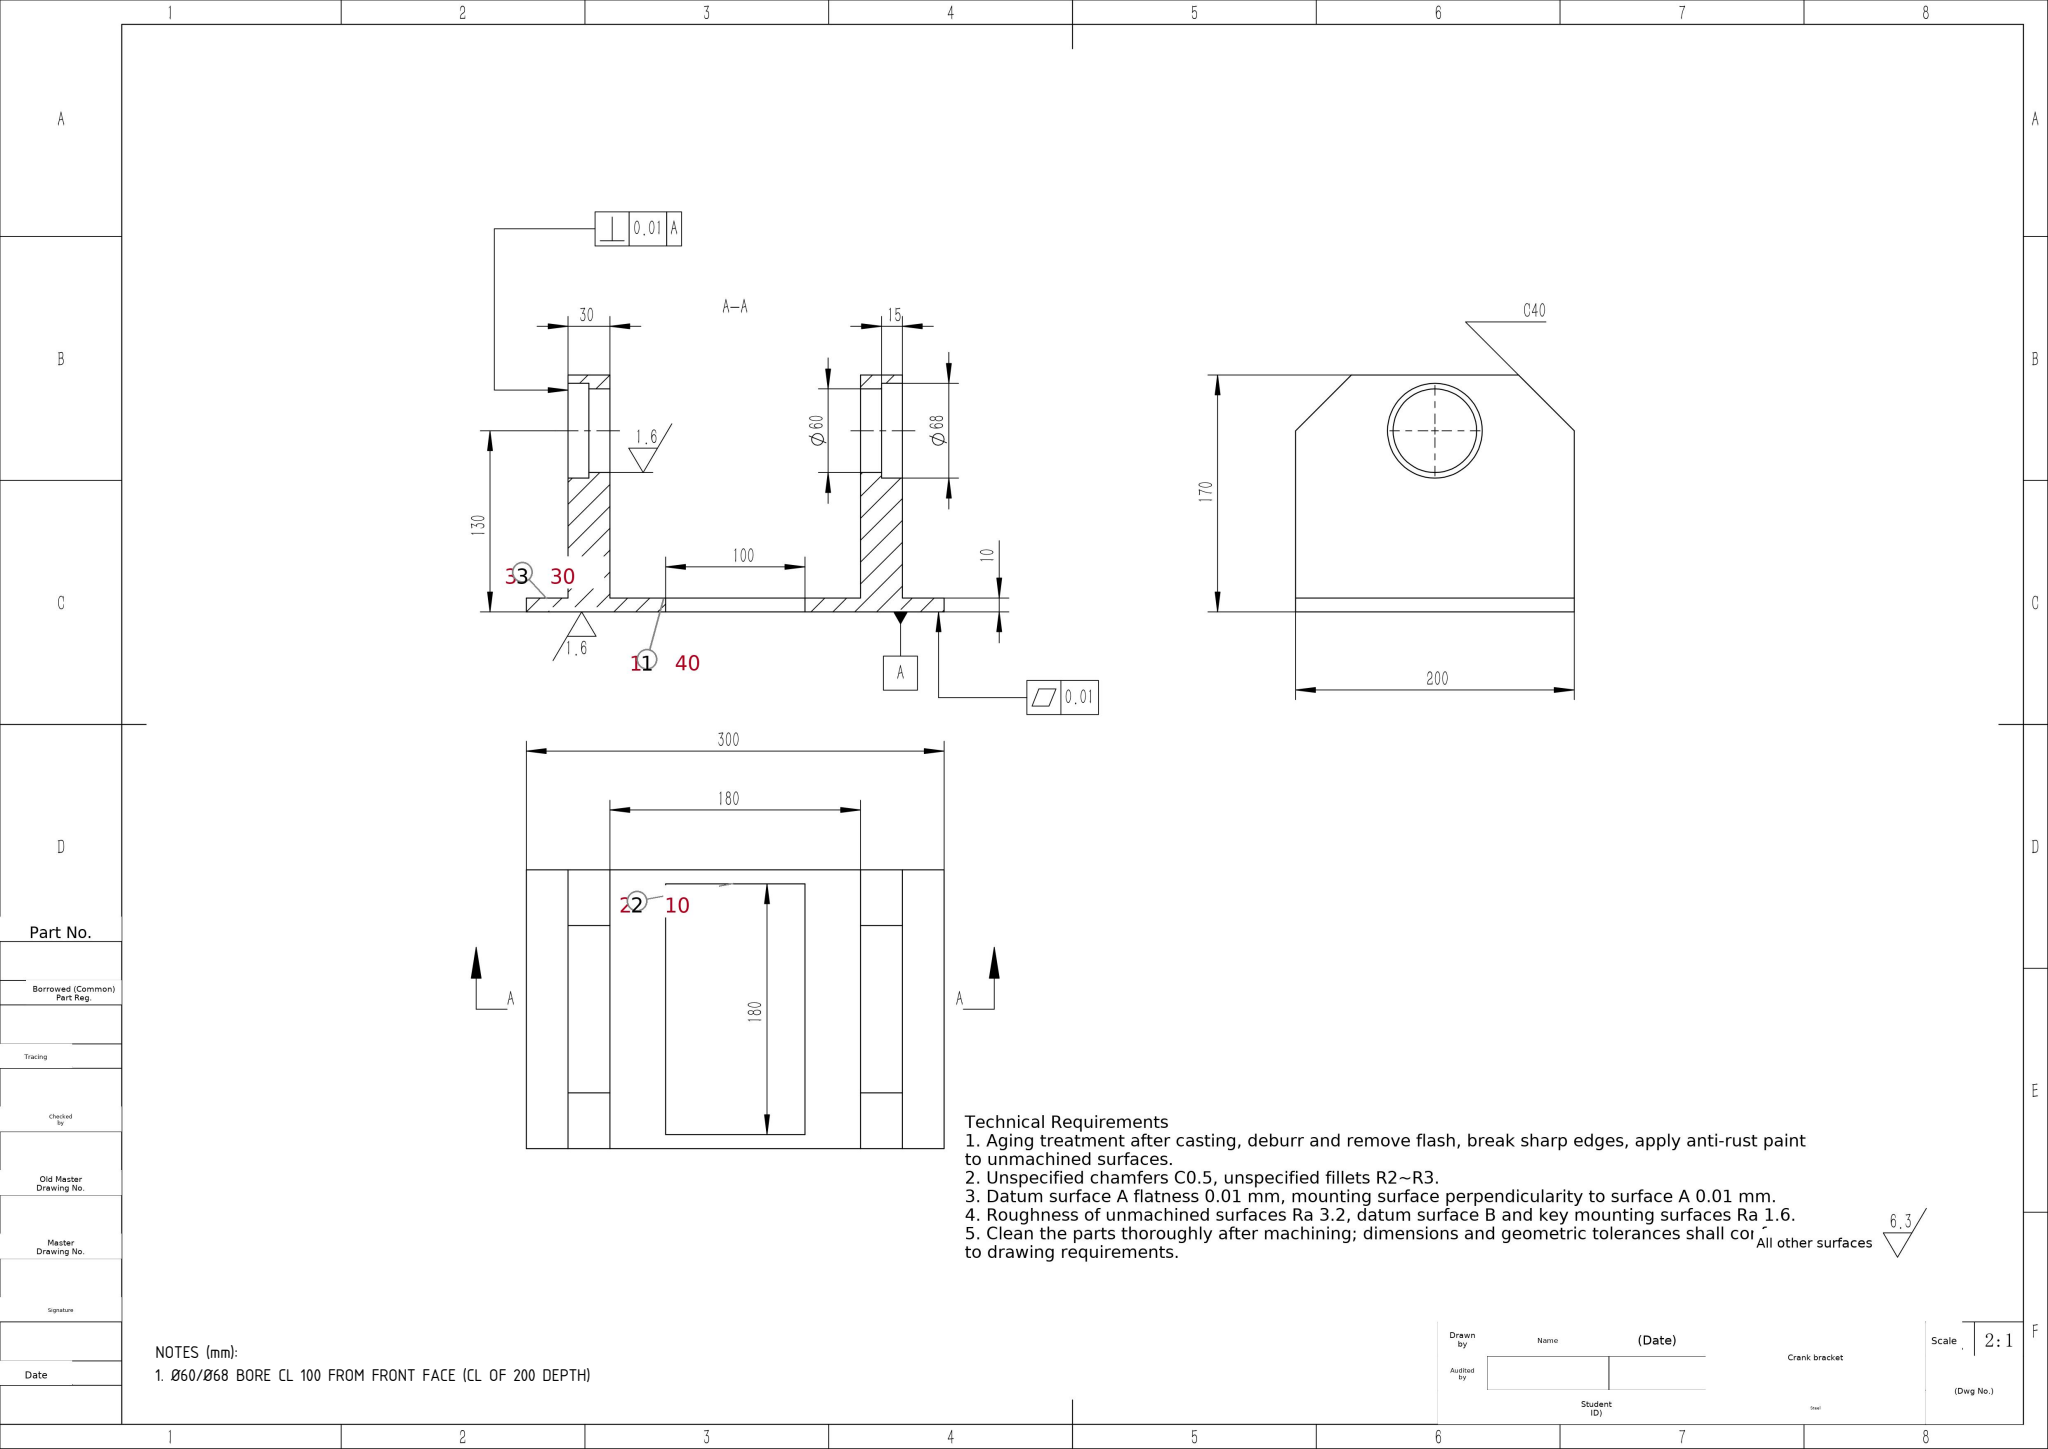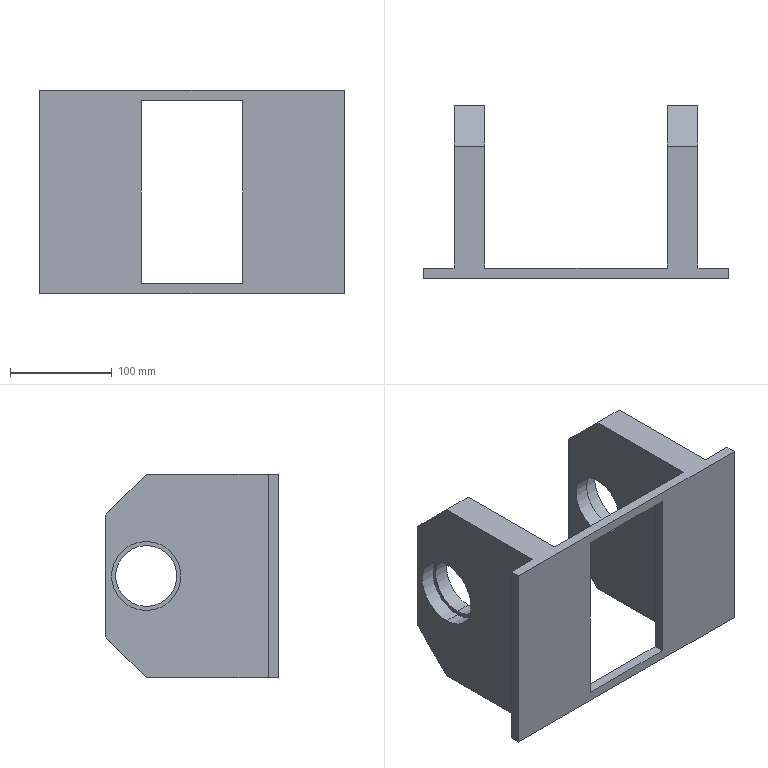Part | SolidWorks | mm | 1 solid | 32 faces | box 300 x 170 x 200 mm | volume 2050227 mm3 | plane 24 | cylinder 8 | commonest cylinder face diameters 68 x4 60 x4
Drawing notes:
Ø60/Ø68 BORE CL 100 FROM FRONT FACE (CL OF 200 DEPTH) | from the solid: cylinders dia 60 & 68, axis x, pos_other_axes [-,130,100]; bbox z=200
build123d program:
from build123d import *

# Parameters (mm, degrees)
SKETCH1_W               = 300
SKETCH1_H               = 200
BOSS_EXTRUDE1_DEPTH     = 10
SKETCH2_W               = 30
SKETCH2_H               = 200
BOSS_EXTRUDE2_DEPTH     = 160
CHAMFER1_SIZE           = 40
CUT_EXTRUDE1_DEPTH      = 377.563
CUT_EXTRUDE1_DEPTH_BACK = 377.563
SKETCH3_R               = 30
SKETCH4_R               = 34
CUT_EXTRUDE2_DEPTH      = 15
CUT_EXTRUDE3_START      = -15
SKETCH5_R               = 34
CUT_EXTRUDE3_DEPTH      = 15
SKETCH6_W               = 100
SKETCH6_H               = 180
CUT_EXTRUDE4_DEPTH      = 395.462


with BuildPart() as part:
    # Sketch1 → Boss-Extrude1 (new body)
    with BuildSketch(Plane(origin=(0, 0, 0), x_dir=(1, 0, 0), z_dir=(0, 1, 0))):
        with Locations((150, 100)):
            Rectangle(SKETCH1_W, SKETCH1_H)
    extrude(amount=BOSS_EXTRUDE1_DEPTH)

    # Sketch2 → Boss-Extrude2 (add)
    with BuildSketch(Plane(origin=(0, 10, 0), x_dir=(1, 0, 0), z_dir=(0, 1, 0))):
        with Locations((45, 100)):
            Rectangle(SKETCH2_W, SKETCH2_H)
        with Locations((255, 100)):
            Rectangle(SKETCH2_W, SKETCH2_H)
    extrude(amount=BOSS_EXTRUDE2_DEPTH)

    # Chamfer1
    chamfer1_edges = [part.edges().sort_by_distance(p)[0] for p in [
        (45, 170, 0),
        (45, 170, -200),
        (255, 170, 0),
        (255, 170, -200),
    ]]
    chamfer(chamfer1_edges, length=CHAMFER1_SIZE)

    # Sketch3 → Cut-Extrude1 (cut, two sides: drawn at the far end of the back side and taken through both)
    with BuildSketch(Plane.ZY.offset(-30).offset(-CUT_EXTRUDE1_DEPTH_BACK)):
        with Locations((-100, 130)):
            Circle(SKETCH3_R)
    extrude(amount=CUT_EXTRUDE1_DEPTH + CUT_EXTRUDE1_DEPTH_BACK, mode=Mode.SUBTRACT)

    # Sketch4 → Cut-Extrude2 (cut)
    with BuildSketch(Plane(origin=(270, 0, 0), x_dir=(0, 0, -1), z_dir=(1, 0, 0))):
        with Locations((100, 130)):
            Circle(SKETCH4_R)
    extrude(amount=-CUT_EXTRUDE2_DEPTH, mode=Mode.SUBTRACT)

    # Sketch5 → Cut-Extrude3 (cut)
    with BuildSketch(Plane.ZY.offset(-30).offset(CUT_EXTRUDE3_START)):
        with Locations(Location((-100, 130, 0), (0, 0, 180))):
            Circle(SKETCH5_R)
    extrude(amount=CUT_EXTRUDE3_DEPTH, mode=Mode.SUBTRACT)

    # Sketch6 → Cut-Extrude4 (cut, through all)
    with BuildSketch(Plane(origin=(0, 10, 0), x_dir=(1, 0, 0), z_dir=(0, 1, 0))):
        with Locations((150, 100)):
            Rectangle(SKETCH6_W, SKETCH6_H)
    extrude(amount=-CUT_EXTRUDE4_DEPTH, mode=Mode.SUBTRACT)


solid = part.part
STEP:
#1=CARTESIAN_POINT('',(45.,130.,-134.));
#2=VERTEX_POINT('',#1);
#3=CARTESIAN_POINT('',(45.,130.,-66.));
#4=VERTEX_POINT('',#3);
#5=CARTESIAN_POINT('',(45.,130.,-100.));
#6=DIRECTION('',(-1.,0.,0.));
#7=DIRECTION('',(0.,0.,1.));
#8=AXIS2_PLACEMENT_3D('',#5,#6,#7);
#9=CIRCLE('',#8,34.);
#10=EDGE_CURVE('',#2,#4,#9,.T.);
#11=ORIENTED_EDGE('',*,*,#10,.F.);
#12=CARTESIAN_POINT('',(30.,130.,-134.));
#13=VERTEX_POINT('',#12);
#14=CARTESIAN_POINT('',(45.,130.,-134.));
#15=DIRECTION('',(-1.,0.,0.));
#16=VECTOR('',#15,1000.);
#17=LINE('',#14,#16);
#18=EDGE_CURVE('',#2,#13,#17,.T.);
#19=ORIENTED_EDGE('',*,*,#18,.T.);
#20=CARTESIAN_POINT('',(30.,130.,-66.));
#21=VERTEX_POINT('',#20);
#22=CARTESIAN_POINT('',(30.,130.,-100.));
#23=DIRECTION('',(-1.,0.,0.));
#24=DIRECTION('',(0.,0.,1.));
#25=AXIS2_PLACEMENT_3D('',#22,#23,#24);
#26=CIRCLE('',#25,34.);
#27=EDGE_CURVE('',#13,#21,#26,.T.);
#28=ORIENTED_EDGE('',*,*,#27,.T.);
#29=CARTESIAN_POINT('',(45.,130.,-66.));
#30=DIRECTION('',(-1.,0.,0.));
#31=VECTOR('',#30,1000.);
#32=LINE('',#29,#31);
#33=EDGE_CURVE('',#4,#21,#32,.T.);
#34=ORIENTED_EDGE('',*,*,#33,.F.);
#35=EDGE_LOOP('',(#11,#19,#28,#34));
#36=FACE_OUTER_BOUND('',#35,.T.);
#37=CARTESIAN_POINT('',(45.,130.,-100.));
#38=DIRECTION('',(-1.,0.,0.));
#39=DIRECTION('',(0.,0.,1.));
#40=AXIS2_PLACEMENT_3D('',#37,#38,#39);
#41=CYLINDRICAL_SURFACE('',#40,34.);
#42=ADVANCED_FACE('',(#36),#41,.F.);
#43=CARTESIAN_POINT('',(255.,130.,-66.));
#44=VERTEX_POINT('',#43);
#45=CARTESIAN_POINT('',(255.,130.,-134.));
#46=VERTEX_POINT('',#45);
#47=CARTESIAN_POINT('',(255.,130.,-100.));
#48=DIRECTION('',(1.,0.,0.));
#49=DIRECTION('',(0.,0.,-1.));
#50=AXIS2_PLACEMENT_3D('',#47,#48,#49);
#51=CIRCLE('',#50,34.);
#52=EDGE_CURVE('',#44,#46,#51,.T.);
#53=ORIENTED_EDGE('',*,*,#52,.F.);
#54=CARTESIAN_POINT('',(270.,130.,-66.));
#55=VERTEX_POINT('',#54);
#56=CARTESIAN_POINT('',(255.,130.,-66.));
#57=DIRECTION('',(1.,0.,0.));
#58=VECTOR('',#57,1000.);
#59=LINE('',#56,#58);
#60=EDGE_CURVE('',#44,#55,#59,.T.);
#61=ORIENTED_EDGE('',*,*,#60,.T.);
#62=CARTESIAN_POINT('',(270.,130.,-134.));
#63=VERTEX_POINT('',#62);
#64=CARTESIAN_POINT('',(270.,130.,-100.));
#65=DIRECTION('',(1.,0.,0.));
#66=DIRECTION('',(0.,0.,-1.));
#67=AXIS2_PLACEMENT_3D('',#64,#65,#66);
#68=CIRCLE('',#67,34.);
#69=EDGE_CURVE('',#55,#63,#68,.T.);
#70=ORIENTED_EDGE('',*,*,#69,.T.);
#71=CARTESIAN_POINT('',(255.,130.,-134.));
#72=DIRECTION('',(1.,0.,0.));
#73=VECTOR('',#72,1000.);
#74=LINE('',#71,#73);
#75=EDGE_CURVE('',#46,#63,#74,.T.);
#76=ORIENTED_EDGE('',*,*,#75,.F.);
#77=EDGE_LOOP('',(#53,#61,#70,#76));
#78=FACE_OUTER_BOUND('',#77,.T.);
#79=CARTESIAN_POINT('',(255.,130.,-100.));
#80=DIRECTION('',(1.,0.,0.));
#81=DIRECTION('',(0.,0.,-1.));
#82=AXIS2_PLACEMENT_3D('',#79,#80,#81);
#83=CYLINDRICAL_SURFACE('',#82,34.);
#84=ADVANCED_FACE('',(#78),#83,.F.);
#85=CARTESIAN_POINT('',(255.,130.,-130.));
#86=VERTEX_POINT('',#85);
#87=CARTESIAN_POINT('',(255.,130.,-70.));
#88=VERTEX_POINT('',#87);
#89=CARTESIAN_POINT('',(255.,130.,-100.));
#90=DIRECTION('',(-1.,0.,0.));
#91=DIRECTION('',(0.,0.,-1.));
#92=AXIS2_PLACEMENT_3D('',#89,#90,#91);
#93=CIRCLE('',#92,30.);
#94=EDGE_CURVE('',#86,#88,#93,.T.);
#95=ORIENTED_EDGE('',*,*,#94,.F.);
#96=CARTESIAN_POINT('',(240.,130.,-130.));
#97=VERTEX_POINT('',#96);
#98=CARTESIAN_POINT('',(300.,130.,-130.));
#99=DIRECTION('',(-1.,0.,0.));
#100=VECTOR('',#99,1000.);
#101=LINE('',#98,#100);
#102=EDGE_CURVE('',#86,#97,#101,.T.);
#103=ORIENTED_EDGE('',*,*,#102,.T.);
#104=CARTESIAN_POINT('',(240.,130.,-70.));
#105=VERTEX_POINT('',#104);
#106=CARTESIAN_POINT('',(240.,130.,-100.));
#107=DIRECTION('',(1.,0.,-0.));
#108=DIRECTION('',(0.,0.,-1.));
#109=AXIS2_PLACEMENT_3D('',#106,#107,#108);
#110=CIRCLE('',#109,30.);
#111=EDGE_CURVE('',#105,#97,#110,.T.);
#112=ORIENTED_EDGE('',*,*,#111,.F.);
#113=CARTESIAN_POINT('',(300.,130.,-70.));
#114=DIRECTION('',(-1.,0.,0.));
#115=VECTOR('',#114,1000.);
#116=LINE('',#113,#115);
#117=EDGE_CURVE('',#88,#105,#116,.T.);
#118=ORIENTED_EDGE('',*,*,#117,.F.);
#119=EDGE_LOOP('',(#95,#103,#112,#118));
#120=FACE_OUTER_BOUND('',#119,.T.);
#121=CARTESIAN_POINT('',(300.,130.,-100.));
#122=DIRECTION('',(-1.,0.,0.));
#123=DIRECTION('',(0.,0.,1.));
#124=AXIS2_PLACEMENT_3D('',#121,#122,#123);
#125=CYLINDRICAL_SURFACE('',#124,30.);
#126=ADVANCED_FACE('',(#120),#125,.F.);
#127=CARTESIAN_POINT('',(60.,130.,-130.));
#128=VERTEX_POINT('',#127);
#129=CARTESIAN_POINT('',(60.,130.,-70.));
#130=VERTEX_POINT('',#129);
#131=CARTESIAN_POINT('',(60.,130.,-100.));
#132=DIRECTION('',(-1.,0.,0.));
#133=DIRECTION('',(0.,0.,1.));
#134=AXIS2_PLACEMENT_3D('',#131,#132,#133);
#135=CIRCLE('',#134,30.);
#136=EDGE_CURVE('',#128,#130,#135,.T.);
#137=ORIENTED_EDGE('',*,*,#136,.F.);
#138=CARTESIAN_POINT('',(45.,130.,-130.));
#139=VERTEX_POINT('',#138);
#140=CARTESIAN_POINT('',(300.,130.,-130.));
#141=DIRECTION('',(-1.,0.,0.));
#142=VECTOR('',#141,1000.);
#143=LINE('',#140,#142);
#144=EDGE_CURVE('',#128,#139,#143,.T.);
#145=ORIENTED_EDGE('',*,*,#144,.T.);
#146=CARTESIAN_POINT('',(45.,130.,-70.));
#147=VERTEX_POINT('',#146);
#148=CARTESIAN_POINT('',(45.,130.,-100.));
#149=DIRECTION('',(1.,0.,-0.));
#150=DIRECTION('',(0.,0.,1.));
#151=AXIS2_PLACEMENT_3D('',#148,#149,#150);
#152=CIRCLE('',#151,30.);
#153=EDGE_CURVE('',#147,#139,#152,.T.);
#154=ORIENTED_EDGE('',*,*,#153,.F.);
#155=CARTESIAN_POINT('',(300.,130.,-70.));
#156=DIRECTION('',(-1.,0.,0.));
#157=VECTOR('',#156,1000.);
#158=LINE('',#155,#157);
#159=EDGE_CURVE('',#130,#147,#158,.T.);
#160=ORIENTED_EDGE('',*,*,#159,.F.);
#161=EDGE_LOOP('',(#137,#145,#154,#160));
#162=FACE_OUTER_BOUND('',#161,.T.);
#163=CARTESIAN_POINT('',(300.,130.,-100.));
#164=DIRECTION('',(-1.,0.,0.));
#165=DIRECTION('',(0.,0.,1.));
#166=AXIS2_PLACEMENT_3D('',#163,#164,#165);
#167=CYLINDRICAL_SURFACE('',#166,30.);
#168=ADVANCED_FACE('',(#162),#167,.F.);
#169=ORIENTED_EDGE('',*,*,#144,.F.);
#170=CARTESIAN_POINT('',(60.,130.,-100.));
#171=DIRECTION('',(-1.,0.,0.));
#172=DIRECTION('',(0.,0.,1.));
#173=AXIS2_PLACEMENT_3D('',#170,#171,#172);
#174=CIRCLE('',#173,30.);
#175=EDGE_CURVE('',#130,#128,#174,.T.);
#176=ORIENTED_EDGE('',*,*,#175,.F.);
#177=ORIENTED_EDGE('',*,*,#159,.T.);
#178=CARTESIAN_POINT('',(45.,130.,-100.));
#179=DIRECTION('',(1.,0.,-0.));
#180=DIRECTION('',(0.,0.,1.));
#181=AXIS2_PLACEMENT_3D('',#178,#179,#180);
#182=CIRCLE('',#181,30.);
#183=EDGE_CURVE('',#139,#147,#182,.T.);
#184=ORIENTED_EDGE('',*,*,#183,.F.);
#185=EDGE_LOOP('',(#169,#176,#177,#184));
#186=FACE_OUTER_BOUND('',#185,.T.);
#187=CARTESIAN_POINT('',(300.,130.,-100.));
#188=DIRECTION('',(-1.,0.,0.));
#189=DIRECTION('',(0.,0.,1.));
#190=AXIS2_PLACEMENT_3D('',#187,#188,#189);
#191=CYLINDRICAL_SURFACE('',#190,30.);
#192=ADVANCED_FACE('',(#186),#191,.F.);
#193=ORIENTED_EDGE('',*,*,#102,.F.);
#194=CARTESIAN_POINT('',(255.,130.,-100.));
#195=DIRECTION('',(-1.,0.,0.));
#196=DIRECTION('',(0.,0.,-1.));
#197=AXIS2_PLACEMENT_3D('',#194,#195,#196);
#198=CIRCLE('',#197,30.);
#199=EDGE_CURVE('',#88,#86,#198,.T.);
#200=ORIENTED_EDGE('',*,*,#199,.F.);
#201=ORIENTED_EDGE('',*,*,#117,.T.);
#202=CARTESIAN_POINT('',(240.,130.,-100.));
#203=DIRECTION('',(1.,0.,-0.));
#204=DIRECTION('',(0.,0.,-1.));
#205=AXIS2_PLACEMENT_3D('',#202,#203,#204);
#206=CIRCLE('',#205,30.);
#207=EDGE_CURVE('',#97,#105,#206,.T.);
#208=ORIENTED_EDGE('',*,*,#207,.F.);
#209=EDGE_LOOP('',(#193,#200,#201,#208));
#210=FACE_OUTER_BOUND('',#209,.T.);
#211=CARTESIAN_POINT('',(300.,130.,-100.));
#212=DIRECTION('',(-1.,0.,0.));
#213=DIRECTION('',(0.,0.,1.));
#214=AXIS2_PLACEMENT_3D('',#211,#212,#213);
#215=CYLINDRICAL_SURFACE('',#214,30.);
#216=ADVANCED_FACE('',(#210),#215,.F.);
#217=CARTESIAN_POINT('',(200.,10.,-190.));
#218=VERTEX_POINT('',#217);
#219=CARTESIAN_POINT('',(100.,10.,-190.));
#220=VERTEX_POINT('',#219);
#221=CARTESIAN_POINT('',(100.,10.,-190.));
#222=DIRECTION('',(-1.,0.,0.));
#223=VECTOR('',#222,1000.);
#224=LINE('',#221,#223);
#225=EDGE_CURVE('',#218,#220,#224,.T.);
#226=ORIENTED_EDGE('',*,*,#225,.F.);
#227=CARTESIAN_POINT('',(200.,10.,-10.));
#228=VERTEX_POINT('',#227);
#229=CARTESIAN_POINT('',(200.,10.,-10.));
#230=DIRECTION('',(0.,0.,-1.));
#231=VECTOR('',#230,1000.);
#232=LINE('',#229,#231);
#233=EDGE_CURVE('',#228,#218,#232,.T.);
#234=ORIENTED_EDGE('',*,*,#233,.F.);
#235=CARTESIAN_POINT('',(100.,10.,-10.));
#236=VERTEX_POINT('',#235);
#237=CARTESIAN_POINT('',(100.,10.,-10.));
#238=DIRECTION('',(1.,0.,0.));
#239=VECTOR('',#238,1000.);
#240=LINE('',#237,#239);
#241=EDGE_CURVE('',#236,#228,#240,.T.);
#242=ORIENTED_EDGE('',*,*,#241,.F.);
#243=CARTESIAN_POINT('',(100.,10.,-10.));
#244=DIRECTION('',(0.,0.,1.));
#245=VECTOR('',#244,1000.);
#246=LINE('',#243,#245);
#247=EDGE_CURVE('',#220,#236,#246,.T.);
#248=ORIENTED_EDGE('',*,*,#247,.F.);
#249=EDGE_LOOP('',(#226,#234,#242,#248));
#250=FACE_BOUND('',#249,.T.);
#251=CARTESIAN_POINT('',(240.,10.,-200.));
#252=VERTEX_POINT('',#251);
#253=CARTESIAN_POINT('',(240.,10.,0.));
#254=VERTEX_POINT('',#253);
#255=CARTESIAN_POINT('',(240.,10.,-200.));
#256=DIRECTION('',(0.,0.,1.));
#257=VECTOR('',#256,1000.);
#258=LINE('',#255,#257);
#259=EDGE_CURVE('',#252,#254,#258,.T.);
#260=ORIENTED_EDGE('',*,*,#259,.F.);
#261=CARTESIAN_POINT('',(60.,10.,-200.));
#262=VERTEX_POINT('',#261);
#263=CARTESIAN_POINT('',(0.,10.,-200.));
#264=DIRECTION('',(-1.,0.,0.));
#265=VECTOR('',#264,1000.);
#266=LINE('',#263,#265);
#267=EDGE_CURVE('',#252,#262,#266,.T.);
#268=ORIENTED_EDGE('',*,*,#267,.T.);
#269=CARTESIAN_POINT('',(60.,10.,0.));
#270=VERTEX_POINT('',#269);
#271=CARTESIAN_POINT('',(60.,10.,-200.));
#272=DIRECTION('',(-0.,0.,-1.));
#273=VECTOR('',#272,1000.);
#274=LINE('',#271,#273);
#275=EDGE_CURVE('',#270,#262,#274,.T.);
#276=ORIENTED_EDGE('',*,*,#275,.F.);
#277=CARTESIAN_POINT('',(0.,10.,0.));
#278=DIRECTION('',(1.,0.,0.));
#279=VECTOR('',#278,1000.);
#280=LINE('',#277,#279);
#281=EDGE_CURVE('',#270,#254,#280,.T.);
#282=ORIENTED_EDGE('',*,*,#281,.T.);
#283=EDGE_LOOP('',(#260,#268,#276,#282));
#284=FACE_OUTER_BOUND('',#283,.T.);
#285=CARTESIAN_POINT('',(0.,10.,0.));
#286=DIRECTION('',(0.,-1.,0.));
#287=DIRECTION('',(0.,0.,-1.));
#288=AXIS2_PLACEMENT_3D('',#285,#286,#287);
#289=PLANE('',#288);
#290=ADVANCED_FACE('',(#250,#284),#289,.F.);
#291=CARTESIAN_POINT('',(270.,10.,0.));
#292=VERTEX_POINT('',#291);
#293=CARTESIAN_POINT('',(270.,10.,-200.));
#294=VERTEX_POINT('',#293);
#295=CARTESIAN_POINT('',(270.,10.,-200.));
#296=DIRECTION('',(0.,0.,-1.));
#297=VECTOR('',#296,1000.);
#298=LINE('',#295,#297);
#299=EDGE_CURVE('',#292,#294,#298,.T.);
#300=ORIENTED_EDGE('',*,*,#299,.F.);
#301=CARTESIAN_POINT('',(300.,10.,0.));
#302=VERTEX_POINT('',#301);
#303=CARTESIAN_POINT('',(0.,10.,0.));
#304=DIRECTION('',(1.,0.,0.));
#305=VECTOR('',#304,1000.);
#306=LINE('',#303,#305);
#307=EDGE_CURVE('',#292,#302,#306,.T.);
#308=ORIENTED_EDGE('',*,*,#307,.T.);
#309=CARTESIAN_POINT('',(300.,10.,-200.));
#310=VERTEX_POINT('',#309);
#311=CARTESIAN_POINT('',(300.,10.,0.));
#312=DIRECTION('',(0.,0.,-1.));
#313=VECTOR('',#312,1000.);
#314=LINE('',#311,#313);
#315=EDGE_CURVE('',#302,#310,#314,.T.);
#316=ORIENTED_EDGE('',*,*,#315,.T.);
#317=CARTESIAN_POINT('',(0.,10.,-200.));
#318=DIRECTION('',(-1.,0.,0.));
#319=VECTOR('',#318,1000.);
#320=LINE('',#317,#319);
#321=EDGE_CURVE('',#310,#294,#320,.T.);
#322=ORIENTED_EDGE('',*,*,#321,.T.);
#323=EDGE_LOOP('',(#300,#308,#316,#322));
#324=FACE_OUTER_BOUND('',#323,.T.);
#325=CARTESIAN_POINT('',(0.,10.,0.));
#326=DIRECTION('',(0.,-1.,0.));
#327=DIRECTION('',(0.,0.,-1.));
#328=AXIS2_PLACEMENT_3D('',#325,#326,#327);
#329=PLANE('',#328);
#330=ADVANCED_FACE('',(#324),#329,.F.);
#331=CARTESIAN_POINT('',(30.,10.,-200.));
#332=VERTEX_POINT('',#331);
#333=CARTESIAN_POINT('',(30.,10.,0.));
#334=VERTEX_POINT('',#333);
#335=CARTESIAN_POINT('',(30.,10.,-200.));
#336=DIRECTION('',(0.,0.,1.));
#337=VECTOR('',#336,1000.);
#338=LINE('',#335,#337);
#339=EDGE_CURVE('',#332,#334,#338,.T.);
#340=ORIENTED_EDGE('',*,*,#339,.F.);
#341=CARTESIAN_POINT('',(0.,10.,-200.));
#342=VERTEX_POINT('',#341);
#343=CARTESIAN_POINT('',(0.,10.,-200.));
#344=DIRECTION('',(-1.,0.,0.));
#345=VECTOR('',#344,1000.);
#346=LINE('',#343,#345);
#347=EDGE_CURVE('',#332,#342,#346,.T.);
#348=ORIENTED_EDGE('',*,*,#347,.T.);
#349=CARTESIAN_POINT('',(0.,10.,0.));
#350=VERTEX_POINT('',#349);
#351=CARTESIAN_POINT('',(0.,10.,0.));
#352=DIRECTION('',(0.,0.,1.));
#353=VECTOR('',#352,1000.);
#354=LINE('',#351,#353);
#355=EDGE_CURVE('',#342,#350,#354,.T.);
#356=ORIENTED_EDGE('',*,*,#355,.T.);
#357=CARTESIAN_POINT('',(0.,10.,0.));
#358=DIRECTION('',(1.,0.,0.));
#359=VECTOR('',#358,1000.);
#360=LINE('',#357,#359);
#361=EDGE_CURVE('',#350,#334,#360,.T.);
#362=ORIENTED_EDGE('',*,*,#361,.T.);
#363=EDGE_LOOP('',(#340,#348,#356,#362));
#364=FACE_OUTER_BOUND('',#363,.T.);
#365=CARTESIAN_POINT('',(0.,10.,0.));
#366=DIRECTION('',(0.,-1.,0.));
#367=DIRECTION('',(0.,0.,-1.));
#368=AXIS2_PLACEMENT_3D('',#365,#366,#367);
#369=PLANE('',#368);
#370=ADVANCED_FACE('',(#364),#369,.F.);
#371=CARTESIAN_POINT('',(0.,0.,-200.));
#372=VERTEX_POINT('',#371);
#373=CARTESIAN_POINT('',(0.,0.,0.));
#374=VERTEX_POINT('',#373);
#375=CARTESIAN_POINT('',(0.,0.,0.));
#376=DIRECTION('',(0.,0.,1.));
#377=VECTOR('',#376,1000.);
#378=LINE('',#375,#377);
#379=EDGE_CURVE('',#372,#374,#378,.T.);
#380=ORIENTED_EDGE('',*,*,#379,.T.);
#381=CARTESIAN_POINT('',(0.,10.,0.));
#382=DIRECTION('',(0.,-1.,0.));
#383=VECTOR('',#382,1000.);
#384=LINE('',#381,#383);
#385=EDGE_CURVE('',#350,#374,#384,.T.);
#386=ORIENTED_EDGE('',*,*,#385,.F.);
#387=ORIENTED_EDGE('',*,*,#355,.F.);
#388=CARTESIAN_POINT('',(0.,10.,-200.));
#389=DIRECTION('',(0.,-1.,0.));
#390=VECTOR('',#389,1000.);
#391=LINE('',#388,#390);
#392=EDGE_CURVE('',#342,#372,#391,.T.);
#393=ORIENTED_EDGE('',*,*,#392,.T.);
#394=EDGE_LOOP('',(#380,#386,#387,#393));
#395=FACE_OUTER_BOUND('',#394,.T.);
#396=CARTESIAN_POINT('',(0.,10.,0.));
#397=DIRECTION('',(1.,0.,0.));
#398=DIRECTION('',(0.,0.,-1.));
#399=AXIS2_PLACEMENT_3D('',#396,#397,#398);
#400=PLANE('',#399);
#401=ADVANCED_FACE('',(#395),#400,.F.);
#402=CARTESIAN_POINT('',(270.,130.,-0.));
#403=VERTEX_POINT('',#402);
#404=CARTESIAN_POINT('',(270.,170.,-0.));
#405=DIRECTION('',(0.,-1.,0.));
#406=VECTOR('',#405,1000.);
#407=LINE('',#404,#406);
#408=EDGE_CURVE('',#403,#292,#407,.T.);
#409=ORIENTED_EDGE('',*,*,#408,.F.);
#410=CARTESIAN_POINT('',(240.,130.,-0.));
#411=VERTEX_POINT('',#410);
#412=CARTESIAN_POINT('',(240.,130.,0.));
#413=DIRECTION('',(-1.,0.,0.));
#414=VECTOR('',#413,1000.);
#415=LINE('',#412,#414);
#416=EDGE_CURVE('',#403,#411,#415,.T.);
#417=ORIENTED_EDGE('',*,*,#416,.T.);
#418=CARTESIAN_POINT('',(240.,170.,-0.));
#419=DIRECTION('',(0.,-1.,0.));
#420=VECTOR('',#419,1000.);
#421=LINE('',#418,#420);
#422=EDGE_CURVE('',#411,#254,#421,.T.);
#423=ORIENTED_EDGE('',*,*,#422,.T.);
#424=ORIENTED_EDGE('',*,*,#281,.F.);
#425=CARTESIAN_POINT('',(60.,130.,-0.));
#426=VERTEX_POINT('',#425);
#427=CARTESIAN_POINT('',(60.,170.,-0.));
#428=DIRECTION('',(0.,-1.,0.));
#429=VECTOR('',#428,1000.);
#430=LINE('',#427,#429);
#431=EDGE_CURVE('',#426,#270,#430,.T.);
#432=ORIENTED_EDGE('',*,*,#431,.F.);
#433=CARTESIAN_POINT('',(30.,130.,-0.));
#434=VERTEX_POINT('',#433);
#435=CARTESIAN_POINT('',(30.,130.,0.));
#436=DIRECTION('',(-1.,0.,0.));
#437=VECTOR('',#436,1000.);
#438=LINE('',#435,#437);
#439=EDGE_CURVE('',#426,#434,#438,.T.);
#440=ORIENTED_EDGE('',*,*,#439,.T.);
#441=CARTESIAN_POINT('',(30.,170.,-0.));
#442=DIRECTION('',(0.,-1.,0.));
#443=VECTOR('',#442,1000.);
#444=LINE('',#441,#443);
#445=EDGE_CURVE('',#434,#334,#444,.T.);
#446=ORIENTED_EDGE('',*,*,#445,.T.);
#447=ORIENTED_EDGE('',*,*,#361,.F.);
#448=ORIENTED_EDGE('',*,*,#385,.T.);
#449=CARTESIAN_POINT('',(300.,0.,0.));
#450=VERTEX_POINT('',#449);
#451=CARTESIAN_POINT('',(0.,0.,0.));
#452=DIRECTION('',(1.,0.,0.));
#453=VECTOR('',#452,1000.);
#454=LINE('',#451,#453);
#455=EDGE_CURVE('',#374,#450,#454,.T.);
#456=ORIENTED_EDGE('',*,*,#455,.T.);
#457=CARTESIAN_POINT('',(300.,10.,0.));
#458=DIRECTION('',(0.,-1.,0.));
#459=VECTOR('',#458,1000.);
#460=LINE('',#457,#459);
#461=EDGE_CURVE('',#302,#450,#460,.T.);
#462=ORIENTED_EDGE('',*,*,#461,.F.);
#463=ORIENTED_EDGE('',*,*,#307,.F.);
#464=EDGE_LOOP('',(#409,#417,#423,#424,#432,#440,#446,#447,#448,#456,#462,#463));
#465=FACE_OUTER_BOUND('',#464,.T.);
#466=CARTESIAN_POINT('',(0.,10.,0.));
#467=DIRECTION('',(0.,0.,-1.));
#468=DIRECTION('',(-1.,0.,0.));
#469=AXIS2_PLACEMENT_3D('',#466,#467,#468);
#470=PLANE('',#469);
#471=ADVANCED_FACE('',(#465),#470,.F.);
#472=CARTESIAN_POINT('',(300.,0.,-200.));
#473=VERTEX_POINT('',#472);
#474=CARTESIAN_POINT('',(300.,0.,0.));
#475=DIRECTION('',(0.,0.,-1.));
#476=VECTOR('',#475,1000.);
#477=LINE('',#474,#476);
#478=EDGE_CURVE('',#450,#473,#477,.T.);
#479=ORIENTED_EDGE('',*,*,#478,.T.);
#480=CARTESIAN_POINT('',(300.,10.,-200.));
#481=DIRECTION('',(0.,-1.,0.));
#482=VECTOR('',#481,1000.);
#483=LINE('',#480,#482);
#484=EDGE_CURVE('',#310,#473,#483,.T.);
#485=ORIENTED_EDGE('',*,*,#484,.F.);
#486=ORIENTED_EDGE('',*,*,#315,.F.);
#487=ORIENTED_EDGE('',*,*,#461,.T.);
#488=EDGE_LOOP('',(#479,#485,#486,#487));
#489=FACE_OUTER_BOUND('',#488,.T.);
#490=CARTESIAN_POINT('',(300.,10.,0.));
#491=DIRECTION('',(-1.,0.,0.));
#492=DIRECTION('',(0.,0.,1.));
#493=AXIS2_PLACEMENT_3D('',#490,#491,#492);
#494=PLANE('',#493);
#495=ADVANCED_FACE('',(#489),#494,.F.);
#496=CARTESIAN_POINT('',(240.,130.,-200.));
#497=VERTEX_POINT('',#496);
#498=CARTESIAN_POINT('',(240.,170.,-200.));
#499=DIRECTION('',(0.,-1.,0.));
#500=VECTOR('',#499,1000.);
#501=LINE('',#498,#500);
#502=EDGE_CURVE('',#497,#252,#501,.T.);
#503=ORIENTED_EDGE('',*,*,#502,.F.);
#504=CARTESIAN_POINT('',(270.,130.,-200.));
#505=VERTEX_POINT('',#504);
#506=CARTESIAN_POINT('',(270.,130.,-200.));
#507=DIRECTION('',(1.,0.,0.));
#508=VECTOR('',#507,1000.);
#509=LINE('',#506,#508);
#510=EDGE_CURVE('',#497,#505,#509,.T.);
#511=ORIENTED_EDGE('',*,*,#510,.T.);
#512=CARTESIAN_POINT('',(270.,170.,-200.));
#513=DIRECTION('',(0.,-1.,0.));
#514=VECTOR('',#513,1000.);
#515=LINE('',#512,#514);
#516=EDGE_CURVE('',#505,#294,#515,.T.);
#517=ORIENTED_EDGE('',*,*,#516,.T.);
#518=ORIENTED_EDGE('',*,*,#321,.F.);
#519=ORIENTED_EDGE('',*,*,#484,.T.);
#520=CARTESIAN_POINT('',(0.,0.,-200.));
#521=DIRECTION('',(-1.,0.,0.));
#522=VECTOR('',#521,1000.);
#523=LINE('',#520,#522);
#524=EDGE_CURVE('',#473,#372,#523,.T.);
#525=ORIENTED_EDGE('',*,*,#524,.T.);
#526=ORIENTED_EDGE('',*,*,#392,.F.);
#527=ORIENTED_EDGE('',*,*,#347,.F.);
#528=CARTESIAN_POINT('',(30.,130.,-200.));
#529=VERTEX_POINT('',#528);
#530=CARTESIAN_POINT('',(30.,170.,-200.));
#531=DIRECTION('',(0.,-1.,0.));
#532=VECTOR('',#531,1000.);
#533=LINE('',#530,#532);
#534=EDGE_CURVE('',#529,#332,#533,.T.);
#535=ORIENTED_EDGE('',*,*,#534,.F.);
#536=CARTESIAN_POINT('',(60.,130.,-200.));
#537=VERTEX_POINT('',#536);
#538=CARTESIAN_POINT('',(60.,130.,-200.));
#539=DIRECTION('',(1.,0.,0.));
#540=VECTOR('',#539,1000.);
#541=LINE('',#538,#540);
#542=EDGE_CURVE('',#529,#537,#541,.T.);
#543=ORIENTED_EDGE('',*,*,#542,.T.);
#544=CARTESIAN_POINT('',(60.,170.,-200.));
#545=DIRECTION('',(0.,-1.,0.));
#546=VECTOR('',#545,1000.);
#547=LINE('',#544,#546);
#548=EDGE_CURVE('',#537,#262,#547,.T.);
#549=ORIENTED_EDGE('',*,*,#548,.T.);
#550=ORIENTED_EDGE('',*,*,#267,.F.);
#551=EDGE_LOOP('',(#503,#511,#517,#518,#519,#525,#526,#527,#535,#543,#549,#550));
#552=FACE_OUTER_BOUND('',#551,.T.);
#553=CARTESIAN_POINT('',(0.,10.,-200.));
#554=DIRECTION('',(0.,0.,1.));
#555=DIRECTION('',(1.,0.,0.));
#556=AXIS2_PLACEMENT_3D('',#553,#554,#555);
#557=PLANE('',#556);
#558=ADVANCED_FACE('',(#552),#557,.F.);
#559=CARTESIAN_POINT('',(200.,0.,-10.));
#560=VERTEX_POINT('',#559);
#561=CARTESIAN_POINT('',(200.,0.,-190.));
#562=VERTEX_POINT('',#561);
#563=CARTESIAN_POINT('',(200.,0.,-10.));
#564=DIRECTION('',(0.,0.,-1.));
#565=VECTOR('',#564,1000.);
#566=LINE('',#563,#565);
#567=EDGE_CURVE('',#560,#562,#566,.T.);
#568=ORIENTED_EDGE('',*,*,#567,.T.);
#569=CARTESIAN_POINT('',(100.,0.,-190.));
#570=VERTEX_POINT('',#569);
#571=CARTESIAN_POINT('',(100.,0.,-190.));
#572=DIRECTION('',(-1.,0.,0.));
#573=VECTOR('',#572,1000.);
#574=LINE('',#571,#573);
#575=EDGE_CURVE('',#562,#570,#574,.T.);
#576=ORIENTED_EDGE('',*,*,#575,.T.);
#577=CARTESIAN_POINT('',(100.,0.,-10.));
#578=VERTEX_POINT('',#577);
#579=CARTESIAN_POINT('',(100.,0.,-10.));
#580=DIRECTION('',(0.,0.,1.));
#581=VECTOR('',#580,1000.);
#582=LINE('',#579,#581);
#583=EDGE_CURVE('',#570,#578,#582,.T.);
#584=ORIENTED_EDGE('',*,*,#583,.T.);
#585=CARTESIAN_POINT('',(100.,0.,-10.));
#586=DIRECTION('',(1.,0.,0.));
#587=VECTOR('',#586,1000.);
#588=LINE('',#585,#587);
#589=EDGE_CURVE('',#578,#560,#588,.T.);
#590=ORIENTED_EDGE('',*,*,#589,.T.);
#591=EDGE_LOOP('',(#568,#576,#584,#590));
#592=FACE_BOUND('',#591,.T.);
#593=ORIENTED_EDGE('',*,*,#379,.F.);
#594=ORIENTED_EDGE('',*,*,#524,.F.);
#595=ORIENTED_EDGE('',*,*,#478,.F.);
#596=ORIENTED_EDGE('',*,*,#455,.F.);
#597=EDGE_LOOP('',(#593,#594,#595,#596));
#598=FACE_OUTER_BOUND('',#597,.T.);
#599=CARTESIAN_POINT('',(0.,0.,0.));
#600=DIRECTION('',(0.,-1.,0.));
#601=DIRECTION('',(0.,0.,-1.));
#602=AXIS2_PLACEMENT_3D('',#599,#600,#601);
#603=PLANE('',#602);
#604=ADVANCED_FACE('',(#592,#598),#603,.T.);
#605=CARTESIAN_POINT('',(30.,130.,-100.));
#606=DIRECTION('',(-1.,0.,0.));
#607=DIRECTION('',(0.,0.,1.));
#608=AXIS2_PLACEMENT_3D('',#605,#606,#607);
#609=CIRCLE('',#608,34.);
#610=EDGE_CURVE('',#21,#13,#609,.T.);
#611=ORIENTED_EDGE('',*,*,#610,.F.);
#612=ORIENTED_EDGE('',*,*,#27,.F.);
#613=EDGE_LOOP('',(#611,#612));
#614=FACE_BOUND('',#613,.T.);
#615=CARTESIAN_POINT('',(30.,170.,-160.));
#616=VERTEX_POINT('',#615);
#617=CARTESIAN_POINT('',(30.,170.,-40.));
#618=VERTEX_POINT('',#617);
#619=CARTESIAN_POINT('',(30.,170.,-200.));
#620=DIRECTION('',(0.,0.,1.));
#621=VECTOR('',#620,1000.);
#622=LINE('',#619,#621);
#623=EDGE_CURVE('',#616,#618,#622,.T.);
#624=ORIENTED_EDGE('',*,*,#623,.F.);
#625=CARTESIAN_POINT('',(30.,170.,-160.));
#626=DIRECTION('',(-0.,-0.7071,-0.7071));
#627=VECTOR('',#626,1000.);
#628=LINE('',#625,#627);
#629=EDGE_CURVE('',#616,#529,#628,.T.);
#630=ORIENTED_EDGE('',*,*,#629,.T.);
#631=ORIENTED_EDGE('',*,*,#534,.T.);
#632=ORIENTED_EDGE('',*,*,#339,.T.);
#633=ORIENTED_EDGE('',*,*,#445,.F.);
#634=CARTESIAN_POINT('',(30.,170.,-40.));
#635=DIRECTION('',(-0.,0.7071,-0.7071));
#636=VECTOR('',#635,1000.);
#637=LINE('',#634,#636);
#638=EDGE_CURVE('',#434,#618,#637,.T.);
#639=ORIENTED_EDGE('',*,*,#638,.T.);
#640=EDGE_LOOP('',(#624,#630,#631,#632,#633,#639));
#641=FACE_OUTER_BOUND('',#640,.T.);
#642=CARTESIAN_POINT('',(30.,170.,-200.));
#643=DIRECTION('',(1.,0.,-0.));
#644=DIRECTION('',(-0.,0.,-1.));
#645=AXIS2_PLACEMENT_3D('',#642,#643,#644);
#646=PLANE('',#645);
#647=ADVANCED_FACE('',(#614,#641),#646,.F.);
#648=ORIENTED_EDGE('',*,*,#175,.T.);
#649=ORIENTED_EDGE('',*,*,#136,.T.);
#650=EDGE_LOOP('',(#648,#649));
#651=FACE_BOUND('',#650,.T.);
#652=ORIENTED_EDGE('',*,*,#548,.F.);
#653=CARTESIAN_POINT('',(60.,170.,-160.));
#654=VERTEX_POINT('',#653);
#655=CARTESIAN_POINT('',(60.,170.,-160.));
#656=DIRECTION('',(0.,0.7071,0.7071));
#657=VECTOR('',#656,1000.);
#658=LINE('',#655,#657);
#659=EDGE_CURVE('',#537,#654,#658,.T.);
#660=ORIENTED_EDGE('',*,*,#659,.T.);
#661=CARTESIAN_POINT('',(60.,170.,-40.));
#662=VERTEX_POINT('',#661);
#663=CARTESIAN_POINT('',(60.,170.,-200.));
#664=DIRECTION('',(-0.,0.,-1.));
#665=VECTOR('',#664,1000.);
#666=LINE('',#663,#665);
#667=EDGE_CURVE('',#662,#654,#666,.T.);
#668=ORIENTED_EDGE('',*,*,#667,.F.);
#669=CARTESIAN_POINT('',(60.,170.,-40.));
#670=DIRECTION('',(0.,-0.7071,0.7071));
#671=VECTOR('',#670,1000.);
#672=LINE('',#669,#671);
#673=EDGE_CURVE('',#662,#426,#672,.T.);
#674=ORIENTED_EDGE('',*,*,#673,.T.);
#675=ORIENTED_EDGE('',*,*,#431,.T.);
#676=ORIENTED_EDGE('',*,*,#275,.T.);
#677=EDGE_LOOP('',(#652,#660,#668,#674,#675,#676));
#678=FACE_OUTER_BOUND('',#677,.T.);
#679=CARTESIAN_POINT('',(60.,170.,-200.));
#680=DIRECTION('',(-1.,0.,0.));
#681=DIRECTION('',(0.,0.,1.));
#682=AXIS2_PLACEMENT_3D('',#679,#680,#681);
#683=PLANE('',#682);
#684=ADVANCED_FACE('',(#651,#678),#683,.F.);
#685=ORIENTED_EDGE('',*,*,#667,.T.);
#686=CARTESIAN_POINT('',(30.,170.,-160.));
#687=DIRECTION('',(-1.,0.,0.));
#688=VECTOR('',#687,1000.);
#689=LINE('',#686,#688);
#690=EDGE_CURVE('',#654,#616,#689,.T.);
#691=ORIENTED_EDGE('',*,*,#690,.T.);
#692=ORIENTED_EDGE('',*,*,#623,.T.);
#693=CARTESIAN_POINT('',(60.,170.,-40.));
#694=DIRECTION('',(1.,0.,0.));
#695=VECTOR('',#694,1000.);
#696=LINE('',#693,#695);
#697=EDGE_CURVE('',#618,#662,#696,.T.);
#698=ORIENTED_EDGE('',*,*,#697,.T.);
#699=EDGE_LOOP('',(#685,#691,#692,#698));
#700=FACE_OUTER_BOUND('',#699,.T.);
#701=CARTESIAN_POINT('',(0.,170.,0.));
#702=DIRECTION('',(0.,1.,0.));
#703=DIRECTION('',(0.,0.,1.));
#704=AXIS2_PLACEMENT_3D('',#701,#702,#703);
#705=PLANE('',#704);
#706=ADVANCED_FACE('',(#700),#705,.T.);
#707=ORIENTED_EDGE('',*,*,#111,.T.);
#708=ORIENTED_EDGE('',*,*,#207,.T.);
#709=EDGE_LOOP('',(#707,#708));
#710=FACE_BOUND('',#709,.T.);
#711=CARTESIAN_POINT('',(240.,170.,-160.));
#712=VERTEX_POINT('',#711);
#713=CARTESIAN_POINT('',(240.,170.,-40.));
#714=VERTEX_POINT('',#713);
#715=CARTESIAN_POINT('',(240.,170.,-200.));
#716=DIRECTION('',(0.,0.,1.));
#717=VECTOR('',#716,1000.);
#718=LINE('',#715,#717);
#719=EDGE_CURVE('',#712,#714,#718,.T.);
#720=ORIENTED_EDGE('',*,*,#719,.F.);
#721=CARTESIAN_POINT('',(240.,170.,-160.));
#722=DIRECTION('',(-0.,-0.7071,-0.7071));
#723=VECTOR('',#722,1000.);
#724=LINE('',#721,#723);
#725=EDGE_CURVE('',#712,#497,#724,.T.);
#726=ORIENTED_EDGE('',*,*,#725,.T.);
#727=ORIENTED_EDGE('',*,*,#502,.T.);
#728=ORIENTED_EDGE('',*,*,#259,.T.);
#729=ORIENTED_EDGE('',*,*,#422,.F.);
#730=CARTESIAN_POINT('',(240.,170.,-40.));
#731=DIRECTION('',(-0.,0.7071,-0.7071));
#732=VECTOR('',#731,1000.);
#733=LINE('',#730,#732);
#734=EDGE_CURVE('',#411,#714,#733,.T.);
#735=ORIENTED_EDGE('',*,*,#734,.T.);
#736=EDGE_LOOP('',(#720,#726,#727,#728,#729,#735));
#737=FACE_OUTER_BOUND('',#736,.T.);
#738=CARTESIAN_POINT('',(240.,170.,-200.));
#739=DIRECTION('',(1.,0.,-0.));
#740=DIRECTION('',(-0.,0.,-1.));
#741=AXIS2_PLACEMENT_3D('',#738,#739,#740);
#742=PLANE('',#741);
#743=ADVANCED_FACE('',(#710,#737),#742,.F.);
#744=CARTESIAN_POINT('',(270.,130.,-100.));
#745=DIRECTION('',(1.,0.,0.));
#746=DIRECTION('',(0.,0.,-1.));
#747=AXIS2_PLACEMENT_3D('',#744,#745,#746);
#748=CIRCLE('',#747,34.);
#749=EDGE_CURVE('',#63,#55,#748,.T.);
#750=ORIENTED_EDGE('',*,*,#749,.F.);
#751=ORIENTED_EDGE('',*,*,#69,.F.);
#752=EDGE_LOOP('',(#750,#751));
#753=FACE_BOUND('',#752,.T.);
#754=ORIENTED_EDGE('',*,*,#516,.F.);
#755=CARTESIAN_POINT('',(270.,170.,-160.));
#756=VERTEX_POINT('',#755);
#757=CARTESIAN_POINT('',(270.,170.,-160.));
#758=DIRECTION('',(0.,0.7071,0.7071));
#759=VECTOR('',#758,1000.);
#760=LINE('',#757,#759);
#761=EDGE_CURVE('',#505,#756,#760,.T.);
#762=ORIENTED_EDGE('',*,*,#761,.T.);
#763=CARTESIAN_POINT('',(270.,170.,-40.));
#764=VERTEX_POINT('',#763);
#765=CARTESIAN_POINT('',(270.,170.,-200.));
#766=DIRECTION('',(0.,0.,-1.));
#767=VECTOR('',#766,1000.);
#768=LINE('',#765,#767);
#769=EDGE_CURVE('',#764,#756,#768,.T.);
#770=ORIENTED_EDGE('',*,*,#769,.F.);
#771=CARTESIAN_POINT('',(270.,170.,-40.));
#772=DIRECTION('',(0.,-0.7071,0.7071));
#773=VECTOR('',#772,1000.);
#774=LINE('',#771,#773);
#775=EDGE_CURVE('',#764,#403,#774,.T.);
#776=ORIENTED_EDGE('',*,*,#775,.T.);
#777=ORIENTED_EDGE('',*,*,#408,.T.);
#778=ORIENTED_EDGE('',*,*,#299,.T.);
#779=EDGE_LOOP('',(#754,#762,#770,#776,#777,#778));
#780=FACE_OUTER_BOUND('',#779,.T.);
#781=CARTESIAN_POINT('',(270.,170.,-200.));
#782=DIRECTION('',(-1.,0.,0.));
#783=DIRECTION('',(0.,0.,1.));
#784=AXIS2_PLACEMENT_3D('',#781,#782,#783);
#785=PLANE('',#784);
#786=ADVANCED_FACE('',(#753,#780),#785,.F.);
#787=ORIENTED_EDGE('',*,*,#769,.T.);
#788=CARTESIAN_POINT('',(240.,170.,-160.));
#789=DIRECTION('',(-1.,0.,0.));
#790=VECTOR('',#789,1000.);
#791=LINE('',#788,#790);
#792=EDGE_CURVE('',#756,#712,#791,.T.);
#793=ORIENTED_EDGE('',*,*,#792,.T.);
#794=ORIENTED_EDGE('',*,*,#719,.T.);
#795=CARTESIAN_POINT('',(270.,170.,-40.));
#796=DIRECTION('',(1.,0.,0.));
#797=VECTOR('',#796,1000.);
#798=LINE('',#795,#797);
#799=EDGE_CURVE('',#714,#764,#798,.T.);
#800=ORIENTED_EDGE('',*,*,#799,.T.);
#801=EDGE_LOOP('',(#787,#793,#794,#800));
#802=FACE_OUTER_BOUND('',#801,.T.);
#803=CARTESIAN_POINT('',(0.,170.,0.));
#804=DIRECTION('',(0.,1.,0.));
#805=DIRECTION('',(0.,0.,1.));
#806=AXIS2_PLACEMENT_3D('',#803,#804,#805);
#807=PLANE('',#806);
#808=ADVANCED_FACE('',(#802),#807,.T.);
#809=ORIENTED_EDGE('',*,*,#761,.F.);
#810=ORIENTED_EDGE('',*,*,#510,.F.);
#811=ORIENTED_EDGE('',*,*,#725,.F.);
#812=ORIENTED_EDGE('',*,*,#792,.F.);
#813=EDGE_LOOP('',(#809,#810,#811,#812));
#814=FACE_OUTER_BOUND('',#813,.T.);
#815=CARTESIAN_POINT('',(0.,170.,-160.));
#816=DIRECTION('',(0.,0.7071,-0.7071));
#817=DIRECTION('',(1.,0.,0.));
#818=AXIS2_PLACEMENT_3D('',#815,#816,#817);
#819=PLANE('',#818);
#820=ADVANCED_FACE('',(#814),#819,.T.);
#821=ORIENTED_EDGE('',*,*,#659,.F.);
#822=ORIENTED_EDGE('',*,*,#542,.F.);
#823=ORIENTED_EDGE('',*,*,#629,.F.);
#824=ORIENTED_EDGE('',*,*,#690,.F.);
#825=EDGE_LOOP('',(#821,#822,#823,#824));
#826=FACE_OUTER_BOUND('',#825,.T.);
#827=CARTESIAN_POINT('',(0.,170.,-160.));
#828=DIRECTION('',(0.,0.7071,-0.7071));
#829=DIRECTION('',(1.,0.,0.));
#830=AXIS2_PLACEMENT_3D('',#827,#828,#829);
#831=PLANE('',#830);
#832=ADVANCED_FACE('',(#826),#831,.T.);
#833=ORIENTED_EDGE('',*,*,#734,.F.);
#834=ORIENTED_EDGE('',*,*,#416,.F.);
#835=ORIENTED_EDGE('',*,*,#775,.F.);
#836=ORIENTED_EDGE('',*,*,#799,.F.);
#837=EDGE_LOOP('',(#833,#834,#835,#836));
#838=FACE_OUTER_BOUND('',#837,.T.);
#839=CARTESIAN_POINT('',(0.,170.,-40.));
#840=DIRECTION('',(0.,0.7071,0.7071));
#841=DIRECTION('',(-1.,0.,0.));
#842=AXIS2_PLACEMENT_3D('',#839,#840,#841);
#843=PLANE('',#842);
#844=ADVANCED_FACE('',(#838),#843,.T.);
#845=ORIENTED_EDGE('',*,*,#638,.F.);
#846=ORIENTED_EDGE('',*,*,#439,.F.);
#847=ORIENTED_EDGE('',*,*,#673,.F.);
#848=ORIENTED_EDGE('',*,*,#697,.F.);
#849=EDGE_LOOP('',(#845,#846,#847,#848));
#850=FACE_OUTER_BOUND('',#849,.T.);
#851=CARTESIAN_POINT('',(0.,170.,-40.));
#852=DIRECTION('',(0.,0.7071,0.7071));
#853=DIRECTION('',(-1.,0.,0.));
#854=AXIS2_PLACEMENT_3D('',#851,#852,#853);
#855=PLANE('',#854);
#856=ADVANCED_FACE('',(#850),#855,.T.);
#857=CARTESIAN_POINT('',(255.,130.,-100.));
#858=DIRECTION('',(1.,0.,0.));
#859=DIRECTION('',(0.,0.,-1.));
#860=AXIS2_PLACEMENT_3D('',#857,#858,#859);
#861=CIRCLE('',#860,34.);
#862=EDGE_CURVE('',#46,#44,#861,.T.);
#863=ORIENTED_EDGE('',*,*,#862,.T.);
#864=ORIENTED_EDGE('',*,*,#52,.T.);
#865=EDGE_LOOP('',(#863,#864));
#866=FACE_OUTER_BOUND('',#865,.T.);
#867=ORIENTED_EDGE('',*,*,#199,.T.);
#868=ORIENTED_EDGE('',*,*,#94,.T.);
#869=EDGE_LOOP('',(#867,#868));
#870=FACE_BOUND('',#869,.T.);
#871=CARTESIAN_POINT('',(255.,130.,-100.));
#872=DIRECTION('',(1.,0.,0.));
#873=DIRECTION('',(0.,0.,-1.));
#874=AXIS2_PLACEMENT_3D('',#871,#872,#873);
#875=PLANE('',#874);
#876=ADVANCED_FACE('',(#866,#870),#875,.T.);
#877=ORIENTED_EDGE('',*,*,#60,.F.);
#878=ORIENTED_EDGE('',*,*,#862,.F.);
#879=ORIENTED_EDGE('',*,*,#75,.T.);
#880=ORIENTED_EDGE('',*,*,#749,.T.);
#881=EDGE_LOOP('',(#877,#878,#879,#880));
#882=FACE_OUTER_BOUND('',#881,.T.);
#883=CARTESIAN_POINT('',(255.,130.,-100.));
#884=DIRECTION('',(1.,0.,0.));
#885=DIRECTION('',(0.,0.,-1.));
#886=AXIS2_PLACEMENT_3D('',#883,#884,#885);
#887=CYLINDRICAL_SURFACE('',#886,34.);
#888=ADVANCED_FACE('',(#882),#887,.F.);
#889=CARTESIAN_POINT('',(45.,130.,-100.));
#890=DIRECTION('',(-1.,0.,0.));
#891=DIRECTION('',(0.,0.,1.));
#892=AXIS2_PLACEMENT_3D('',#889,#890,#891);
#893=CIRCLE('',#892,34.);
#894=EDGE_CURVE('',#4,#2,#893,.T.);
#895=ORIENTED_EDGE('',*,*,#894,.T.);
#896=ORIENTED_EDGE('',*,*,#10,.T.);
#897=EDGE_LOOP('',(#895,#896));
#898=FACE_OUTER_BOUND('',#897,.T.);
#899=ORIENTED_EDGE('',*,*,#153,.T.);
#900=ORIENTED_EDGE('',*,*,#183,.T.);
#901=EDGE_LOOP('',(#899,#900));
#902=FACE_BOUND('',#901,.T.);
#903=CARTESIAN_POINT('',(45.,130.,-100.));
#904=DIRECTION('',(-1.,0.,0.));
#905=DIRECTION('',(0.,0.,1.));
#906=AXIS2_PLACEMENT_3D('',#903,#904,#905);
#907=PLANE('',#906);
#908=ADVANCED_FACE('',(#898,#902),#907,.T.);
#909=ORIENTED_EDGE('',*,*,#18,.F.);
#910=ORIENTED_EDGE('',*,*,#894,.F.);
#911=ORIENTED_EDGE('',*,*,#33,.T.);
#912=ORIENTED_EDGE('',*,*,#610,.T.);
#913=EDGE_LOOP('',(#909,#910,#911,#912));
#914=FACE_OUTER_BOUND('',#913,.T.);
#915=CARTESIAN_POINT('',(45.,130.,-100.));
#916=DIRECTION('',(-1.,0.,0.));
#917=DIRECTION('',(0.,0.,1.));
#918=AXIS2_PLACEMENT_3D('',#915,#916,#917);
#919=CYLINDRICAL_SURFACE('',#918,34.);
#920=ADVANCED_FACE('',(#914),#919,.F.);
#921=ORIENTED_EDGE('',*,*,#233,.T.);
#922=CARTESIAN_POINT('',(200.,0.,-190.));
#923=DIRECTION('',(0.,1.,0.));
#924=VECTOR('',#923,1000.);
#925=LINE('',#922,#924);
#926=EDGE_CURVE('',#562,#218,#925,.T.);
#927=ORIENTED_EDGE('',*,*,#926,.F.);
#928=ORIENTED_EDGE('',*,*,#567,.F.);
#929=CARTESIAN_POINT('',(200.,0.,-10.));
#930=DIRECTION('',(0.,1.,0.));
#931=VECTOR('',#930,1000.);
#932=LINE('',#929,#931);
#933=EDGE_CURVE('',#560,#228,#932,.T.);
#934=ORIENTED_EDGE('',*,*,#933,.T.);
#935=EDGE_LOOP('',(#921,#927,#928,#934));
#936=FACE_OUTER_BOUND('',#935,.T.);
#937=CARTESIAN_POINT('',(200.,0.,-10.));
#938=DIRECTION('',(1.,0.,0.));
#939=DIRECTION('',(0.,0.,-1.));
#940=AXIS2_PLACEMENT_3D('',#937,#938,#939);
#941=PLANE('',#940);
#942=ADVANCED_FACE('',(#936),#941,.F.);
#943=ORIENTED_EDGE('',*,*,#241,.T.);
#944=ORIENTED_EDGE('',*,*,#933,.F.);
#945=ORIENTED_EDGE('',*,*,#589,.F.);
#946=CARTESIAN_POINT('',(100.,0.,-10.));
#947=DIRECTION('',(0.,1.,0.));
#948=VECTOR('',#947,1000.);
#949=LINE('',#946,#948);
#950=EDGE_CURVE('',#578,#236,#949,.T.);
#951=ORIENTED_EDGE('',*,*,#950,.T.);
#952=EDGE_LOOP('',(#943,#944,#945,#951));
#953=FACE_OUTER_BOUND('',#952,.T.);
#954=CARTESIAN_POINT('',(100.,0.,-10.));
#955=DIRECTION('',(0.,0.,1.));
#956=DIRECTION('',(1.,0.,0.));
#957=AXIS2_PLACEMENT_3D('',#954,#955,#956);
#958=PLANE('',#957);
#959=ADVANCED_FACE('',(#953),#958,.F.);
#960=ORIENTED_EDGE('',*,*,#247,.T.);
#961=ORIENTED_EDGE('',*,*,#950,.F.);
#962=ORIENTED_EDGE('',*,*,#583,.F.);
#963=CARTESIAN_POINT('',(100.,0.,-190.));
#964=DIRECTION('',(0.,1.,0.));
#965=VECTOR('',#964,1000.);
#966=LINE('',#963,#965);
#967=EDGE_CURVE('',#570,#220,#966,.T.);
#968=ORIENTED_EDGE('',*,*,#967,.T.);
#969=EDGE_LOOP('',(#960,#961,#962,#968));
#970=FACE_OUTER_BOUND('',#969,.T.);
#971=CARTESIAN_POINT('',(100.,0.,-10.));
#972=DIRECTION('',(-1.,0.,0.));
#973=DIRECTION('',(0.,0.,1.));
#974=AXIS2_PLACEMENT_3D('',#971,#972,#973);
#975=PLANE('',#974);
#976=ADVANCED_FACE('',(#970),#975,.F.);
#977=ORIENTED_EDGE('',*,*,#225,.T.);
#978=ORIENTED_EDGE('',*,*,#967,.F.);
#979=ORIENTED_EDGE('',*,*,#575,.F.);
#980=ORIENTED_EDGE('',*,*,#926,.T.);
#981=EDGE_LOOP('',(#977,#978,#979,#980));
#982=FACE_OUTER_BOUND('',#981,.T.);
#983=CARTESIAN_POINT('',(100.,0.,-190.));
#984=DIRECTION('',(0.,0.,-1.));
#985=DIRECTION('',(-1.,0.,0.));
#986=AXIS2_PLACEMENT_3D('',#983,#984,#985);
#987=PLANE('',#986);
#988=ADVANCED_FACE('',(#982),#987,.F.);
#989=CLOSED_SHELL('',(#42,#84,#126,#168,#192,#216,#290,#330,#370,#401,#471,#495,#558,#604,#647,#684,#706,#743,#786,#808,#820,#832,#844,#856,#876,#888,#908,#920,#942,#959,#976,#988));
#990=MANIFOLD_SOLID_BREP('',#989);
#991=CARTESIAN_POINT('',(0.,0.,0.));
#992=DIRECTION('',(0.,0.,1.));
#993=DIRECTION('',(1.,0.,0.));
#994=AXIS2_PLACEMENT_3D('',#991,#992,#993);
#995=(LENGTH_UNIT()NAMED_UNIT(*)SI_UNIT(.MILLI.,.METRE.));
#996=UNCERTAINTY_MEASURE_WITH_UNIT(LENGTH_MEASURE(0.00001),#995,'','');
#997=(NAMED_UNIT(*)PLANE_ANGLE_UNIT()SI_UNIT($,.RADIAN.));
#998=(NAMED_UNIT(*)SI_UNIT($,.STERADIAN.)SOLID_ANGLE_UNIT());
#999=(GEOMETRIC_REPRESENTATION_CONTEXT(3)GLOBAL_UNCERTAINTY_ASSIGNED_CONTEXT((#996))GLOBAL_UNIT_ASSIGNED_CONTEXT((#995,#997,#998))REPRESENTATION_CONTEXT('',''));
#1000=ADVANCED_BREP_SHAPE_REPRESENTATION('',(#990,#994),#999);